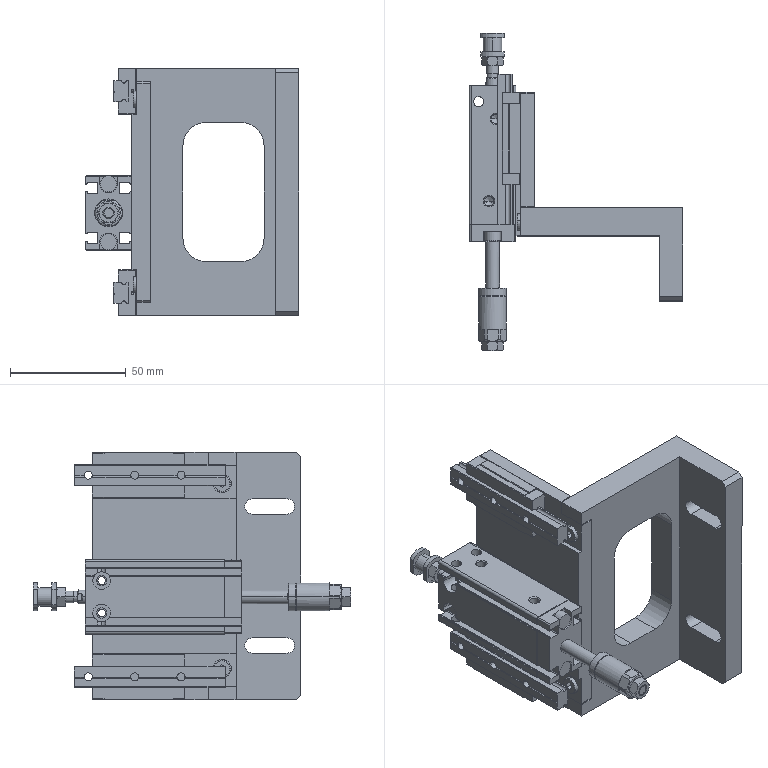Assembly | SolidWorks | mm | 15 component files | 15 solids | 707 faces | box 92.2 x 137 x 107 mm | volume 183868 mm3 | plane 320 | cylinder 282 | cone 91 | torus 12 | spline 2 | commonest cylinder face diameters 0.4 x44 3.5 x28 4.5 x22 6 x20 2 x16 3 x16 0.8 x16 4 x12
Bill of materials:
F01AE00021-D54311 | 1 |  | Flat rectangular plate with a stepped outline and multiple through holes; one long edge has notched corners and a thin raised strip on the back face.
F01AE00021-D54312B | 1 | AL6061 | L-shaped angle bracket. One leg has a large rounded-rectangle cutout, the other leg has two parallel slots, and there is one small hole.
F01AE00021-D54313 | 1 |  | Spool-shaped bushing: a cylindrical body between two end flanges, with a central through bore. The flanges have flats cut on two opposite sides.
MDJ16x20-10S_00_+_1 | 1 |  | Rectangular prismatic block with slot-like grooves running its full length at the corners, a central through bore along its length, and several cross holes on the faces.
MDJ16x20-10S_00_+_2 | 1 |  | Long stepped round shaft with a short larger-diameter cylindrical collar near its middle and reduced-diameter journals at both ends.
MDJ16x20-10S_00_+_3 | 1 |  | Hexagonal nut-shaped body with a round central through bore and chamfered corners on both faces.
MDJ16x20-10S_00_+_4 | 1 |  | Cylindrical sleeve with a central through bore, a short hexagonal section at one end, and a shallow groove around the circumference near the other end.
MDJ16x20-10S_00_+_5 | 1 |  | Hexagonal nut-shaped body with a round central through bore and chamfered corners on both faces.
MGN9-HSlider-D | 2 | 45 | Rectangular block with a C-shaped channel cross-section, rounded relief grooves at the inner corners, four recessed holes on the main face, and separate-looking end sections.
SocketHeadCapScrew_M4_12-D | 3 |  | Headed pin or cap-screw-like body: a cylindrical head, a smaller cylindrical shank with a fillet under the head, and a chamfered tip.
XMGN9C-70GuideRail--D | 2 |  | Long rectangular bar with a semicircular groove along each long side, a small side groove, and three evenly spaced through holes.
Mates:
1. coincident | MGN9-HSlider-D-1 face at (279.434, 97.755, 300.264) dir (0, -1, 0) | MGN9-HSlider-D-2 face at (279.434, 97.755, 213.264) dir (0, -1, 0)
2. coincident | F01AE00021-D54311-1 face at (290.434, 137.705, 193.264) dir (0, 0, -1) | MGN9-HSlider-D-2 face at (276.434, 137.655, 193.264) dir (0, 0, -1)
3. coincident | F01AE00021-D54311-1 face at (290.434, 75.705, 193.264) dir (0, -1, 0) | F01AE00021-D54312B-1 face at (284.434, 75.705, 193.264) dir (0, -1, 0)
4. width | F01AE00021-D54311-1 face at (290.434, 137.705, 193.264) dir (0, 0, -1) | F01AE00021-D54311-1 face at (290.434, 137.705, 300.264) dir (0, 0, 1) | F01AE00021-D54312B-1 face at (354.434, 87.705, 300.264) dir (0, 0, 1) | F01AE00021-D54312B-1 face at (354.434, 87.705, 193.264) dir (0, 0, -1)
5. coincident | F01AE00021-D54311-1 face at (287.034, 81.705, 289.014) dir (-1, 0, 0) | SocketHeadCapScrew_M4_12-D-2 face at (287.034, 85.157, 286.188) dir (1, 0, 0)
6. coincident | SocketHeadCapScrew_M4_12-D-2 face at (287.034, 85.157, 286.188) dir (1, 0, 0) | SocketHeadCapScrew_M4_12-D-3 face at (287.034, 85.157, 206.188) dir (1, 0, 0)
7. coincident | SocketHeadCapScrew_M4_12-D-1 face at (287.034, 85.157, 246.188) dir (1, 0, 0) | SocketHeadCapScrew_M4_12-D-3 face at (287.034, 85.157, 206.188) dir (1, 0, 0)
8. concentric | F01AE00021-D54311-1 edge at (287.034, 81.705, 286.764) dir (-1, 0, 0) r 2.25 | SocketHeadCapScrew_M4_12-D-2 face at (283.034, 81.705, 286.764) dir (-1, 0, 0) r 2
9. concentric | F01AE00021-D54311-1 face at (282.434, 81.705, 206.764) dir (-1, 0, 0) r 2.25 | SocketHeadCapScrew_M4_12-D-3 face at (283.034, 81.705, 206.764) dir (-1, 0, 0) r 2
10. concentric | F01AE00021-D54311-1 face at (282.434, 81.705, 246.764) dir (-1, 0, 0) r 2.25 | SocketHeadCapScrew_M4_12-D-1 face at (283.034, 81.705, 246.764) dir (-1, 0, 0) r 2
11. width | MGN9-HSlider-D-2 face at (276.434, 137.655, 193.264) dir (0, 0, -1) | MGN9-HSlider-D-2 face at (279.134, 137.655, 213.264) dir (0, 0, 1) | XMGN9C-70GuideRail--D-2 face at (277.934, 89.432, 207.764) dir (0, 0, 1) | XMGN9C-70GuideRail--D-2 face at (274.434, 89.432, 198.764) dir (0, 0, -1)
12. coincident | XMGN9C-70GuideRail--D-2 face at (280.934, 89.432, 198.764) dir (1, 0, 0) | MGN9-HSlider-D-2 face at (280.934, 145.205, 207.764) dir (-1, 0, 0)
13. concentric | F01AE00021-D54311-1 face at (290.434, 125.705, 195.764) dir (1, 0, 0) r 1.75 | MGN9-HSlider-D-2 face at (284.434, 125.705, 195.764) dir (-1, 0, 0) r 1.5
14. coincident | F01AE00021-D54311-1 face at (284.434, 206.705, 213.264) dir (-1, 0, 0) | MGN9-HSlider-D-2 face at (284.434, 137.655, 193.264) dir (1, 0, 0)
15. width | XMGN9C-70GuideRail--D-1 face at (277.934, 89.432, 294.764) dir (0, 0, 1) | XMGN9C-70GuideRail--D-1 face at (274.434, 89.432, 285.764) dir (0, 0, -1) | MGN9-HSlider-D-1 face at (276.434, 97.755, 299.964) dir (0, 0, 1) | MGN9-HSlider-D-1 face at (284.134, 97.755, 280.564) dir (0, 0, -1)
16. coincident | F01AE00021-D54311-1 face at (290.434, 106.705, 246.764) dir (1, 0, 0) | F01AE00021-D54312B-1 face at (290.434, 47.705, 199.264) dir (-1, 0, 0)
17. coincident | XMGN9C-70GuideRail--D-1 face at (280.934, 89.432, 285.764) dir (1, 0, 0) | MGN9-HSlider-D-1 face at (280.934, 145.205, 294.764) dir (-1, 0, 0)
18. coincident | F01AE00021-D54311-1 face at (284.434, 206.705, 280.264) dir (-1, 0, 0) | MGN9-HSlider-D-1 face at (284.434, 137.655, 280.264) dir (1, 0, 0)
19. concentric | F01AE00021-D54311-1 face at (290.434, 109.705, 282.764) dir (1, 0, 0) r 1.75 | MGN9-HSlider-D-1 face at (284.434, 109.705, 282.764) dir (-1, 0, 0) r 1.5
20. parallel | F01AE00021-D54312B-1 face at (354.434, 87.705, 193.264) dir (0, 0, -1) | assembly plane at (0, 0, 0) dir (0, 0, 1)
21. concentric | F01AE00021-D54311-1 face at (282.434, 133.705, 230.764) dir (-1, 0, 0) r 1.65 | MDJ16x20-10S_00_+-1/MDJ16x20-10S_00_+_1-1 face at (272.334, 133.705, 230.764) dir (1, 0, 0) r 2.25
22. coincident | F01AE00021-D54311-1 face at (282.434, 106.705, 246.764) dir (-1, 0, 0) | MDJ16x20-10S_00_+-1/MDJ16x20-10S_00_+_1-1 face at (282.434, 140.705, 246.614) dir (1, 0, 0)
23. concentric | F01AE00021-D54311-1 face at (282.434, 133.705, 244.764) dir (-1, 0, 0) r 1.65 | MDJ16x20-10S_00_+-1/MDJ16x20-10S_00_+_1-1 face at (272.334, 133.705, 244.764) dir (1, 0, 0) r 2.25
24. concentric | F01AE00021-D54313-1 face at (272.334, 162.435, 237.764) dir (0, 1, 0) r 2.1 | MDJ16x20-10S_00_+-1/MDJ16x20-10S_00_+_2-1 face at (272.334, 150.96, 237.764) dir (0, -1, 0) r 2.5
25. distance | F01AE00021-D54313-1 face at (274.334, 153.205, 237.764) dir (0, -1, 0) | MDJ16x20-10S_00_+-1/MDJ16x20-10S_00_+_3-1 face at (274.334, 149.205, 237.764) dir (0, -1, 0)
26. parallel | F01AE00021-D54313-1 face at (267.334, 153.205, 234.448) dir (-1, 0, 0) | MDJ16x20-10S_00_+-1/MDJ16x20-10S_00_+_1-1 face at (262.234, 140.705, 228.914) dir (-1, 0, 0)